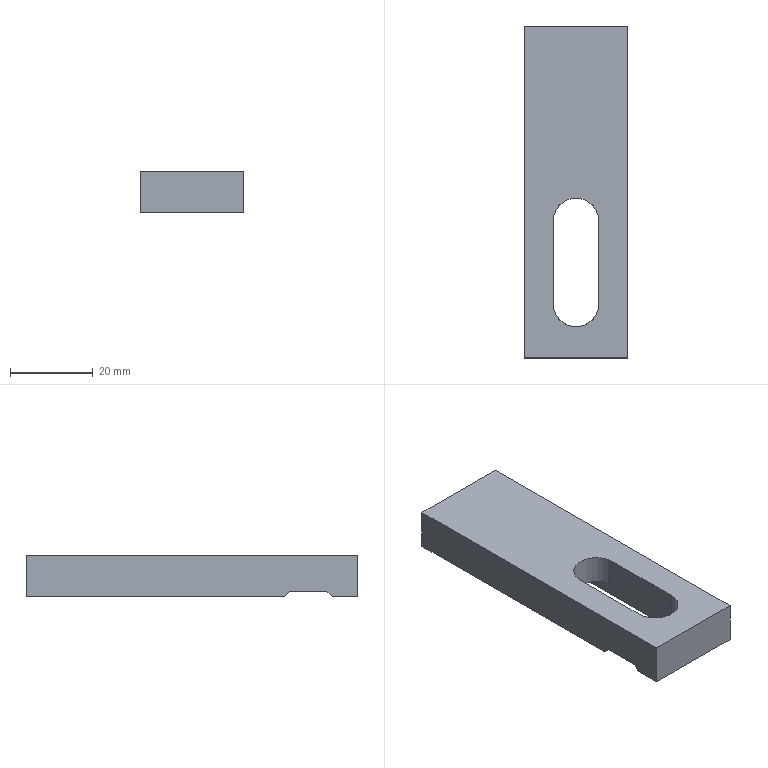Component | NX | CLAMPING_PLATE | 1 solid | 18 faces | volume 15228 mm3 | plane 16 | cylinder 2 | commonest cylinder face diameters 11 x2